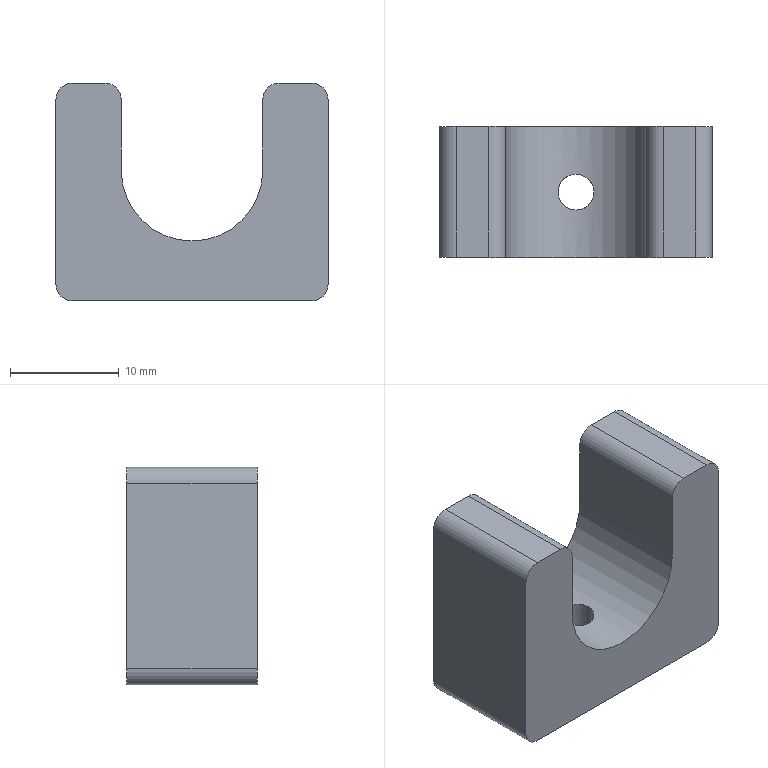CAM job | Mastercam | mm | 7 operations | part box 25 x 12 x 20
1. Facing | 20 - 63 平铣刀
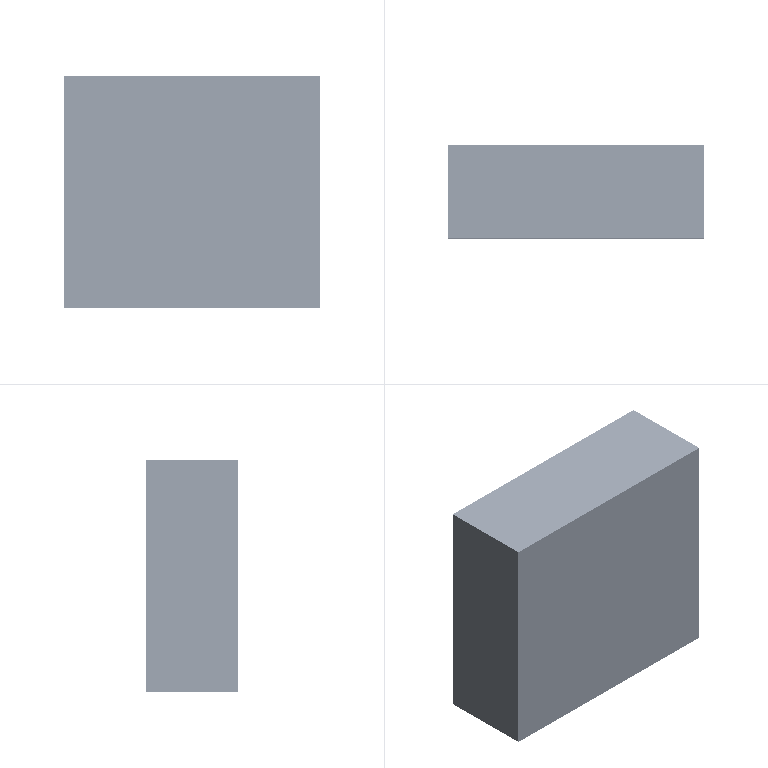2. 2D High Speed (2D Dynamic Mill) | 8 - 8 平铣刀
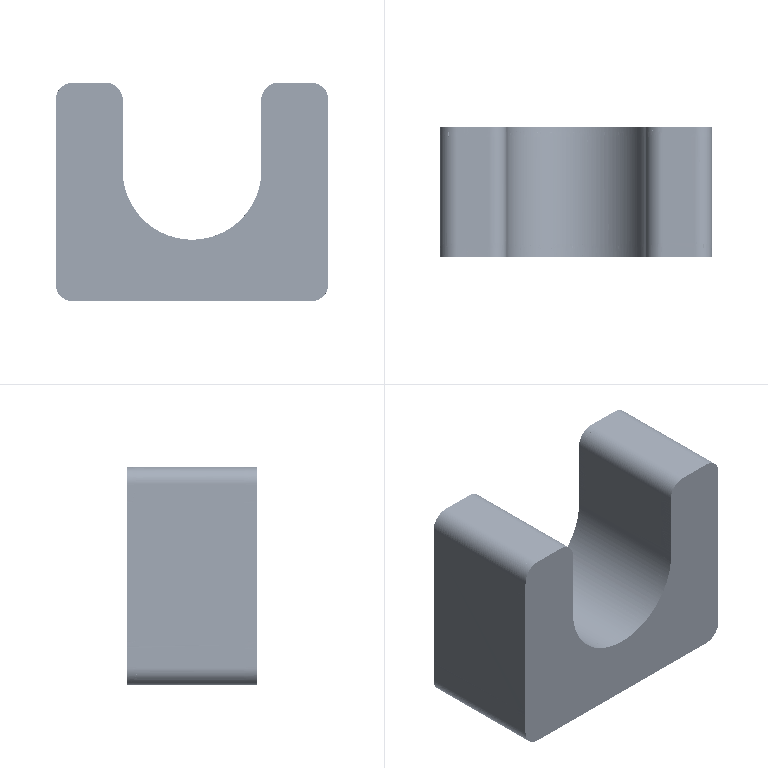3. Contour (2D) | 8 - 8 平铣刀
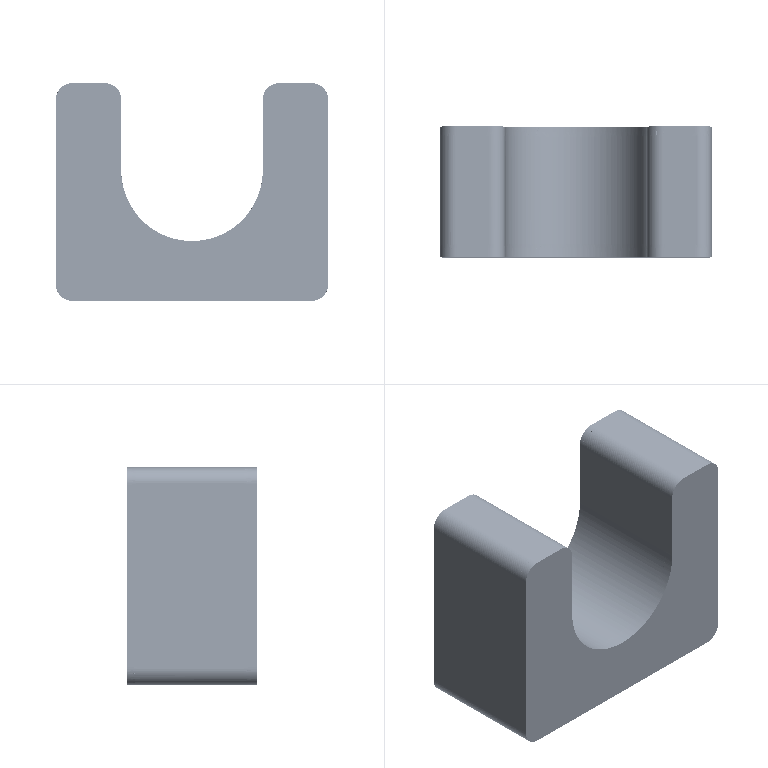4. Contour (2D chamfer) | 7 - 4 倒角刀
5. Facing | 20 - 63 平铣刀
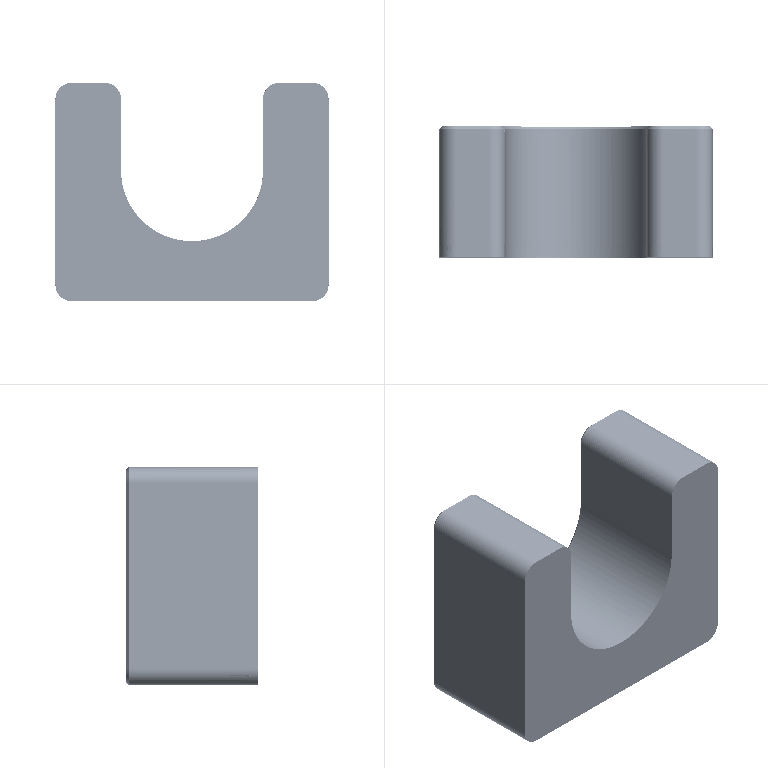6. Contour (2D chamfer) | 7 - 4 倒角刀
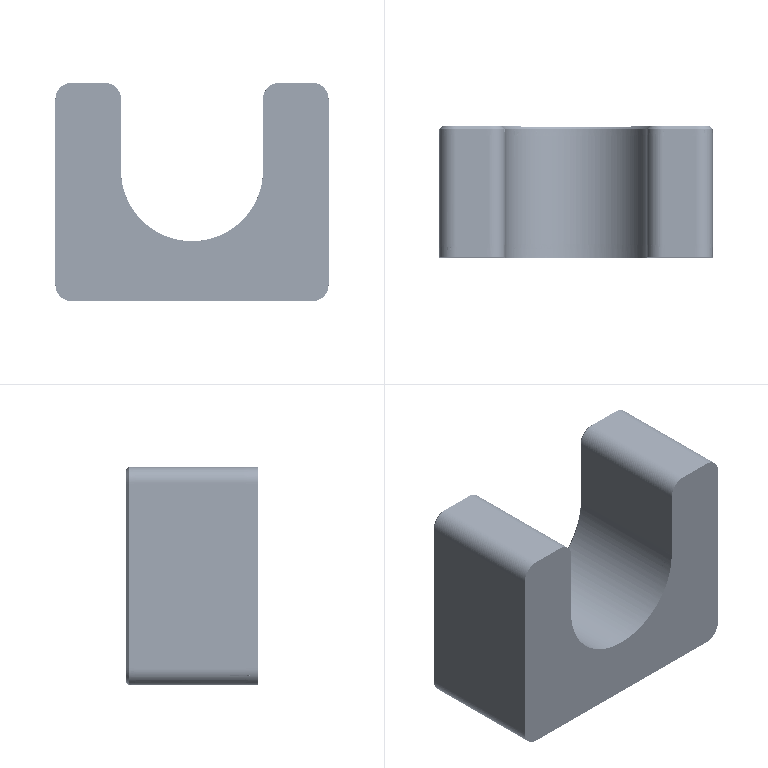7. Drill/Counterbore | 7 - 4 倒角刀